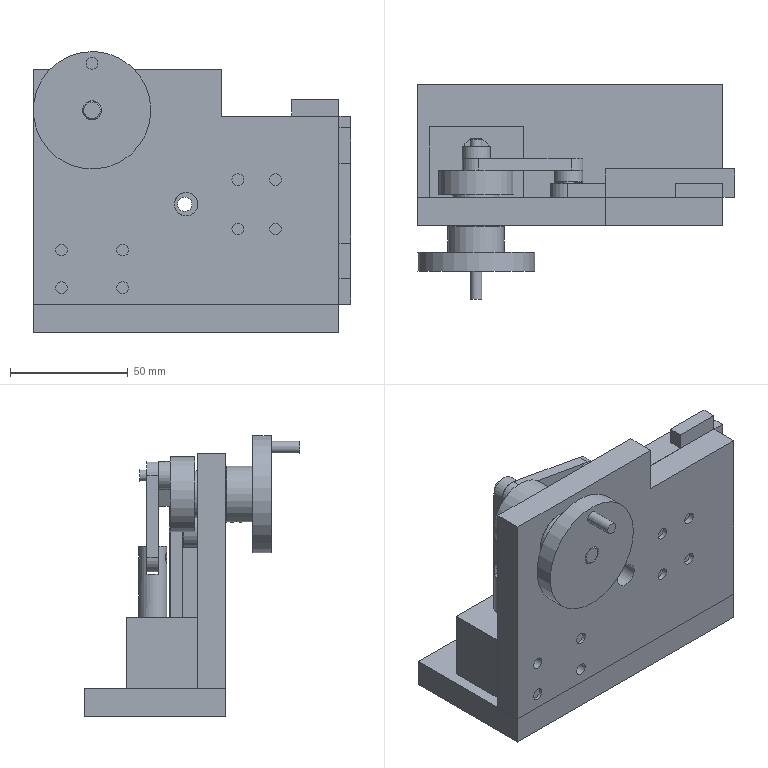Assembly | NX | mm | 27 component files | 27 solids | 262 faces | box 135 x 91.5 x 119.5 mm | volume 362094 mm3 | plane 174 | cylinder 82 | cone 6 | commonest cylinder face diameters 5 x36 12 x9 5.5 x8 10 x7 5.1 x6 8.28 x4 8 x2 6.1 x2
Bill of materials:
unnamed part 1 | 1 |  | Rectangular plate-like block with a stepped profile: raised rails/tabs and rectangular notches along its edges, a rectangular recess on one side, and four round holes in a 2x2 pattern on one region of the face.
unnamed part 2 | 1 |  | Thin flat plate of uniform thickness. One long edge is straight and the opposite edge has two V-shaped notches, giving it a sawtooth-like outline.
unnamed part 3 | 6 |  | Plain solid cylinder (round rod segment) with flat ends.
unnamed part 4 | 2 |  | Stepped cylindrical pin: a short, larger-diameter cylindrical head joined coaxially to a longer, smaller-diameter cylindrical shaft, with a flat shoulder between them.
unnamed part 5 | 1 |  | Rectangular block with one larger round hole through one face and four smaller round holes in a rectangular pattern on an adjacent face.
unnamed part 6 | 1 |  | Flanged disc: a large thin circular flange with a smaller coaxial cylindrical boss on one side. It has a central round through hole and one smaller round hole offset near the edge of the flange.
unnamed part 7 | 2 |  | Flat bar of uniform thickness with one semicircular rounded end containing a round through hole. The opposite end is pointed (chevron-shaped).
unnamed part 8 | 3 |  | Plain solid cylinder with flat ends, relatively short and wide compared with unnamed part 3.
unnamed part 9 | 1 |  | Cylinder with a conical pointed top and a rectangular slot cut into the bottom edge on one side.
unnamed part 10 | 1 |  | Flat plate of uniform thickness with a stepped outline: a rectangular portion is cut away at one corner. It has two larger round holes and two groups of four smaller round holes, each group arranged in a square or rectangular pattern.
unnamed part 11 | 1 |  | Cylindrical pin with a fork-like slotted end: a straight slot across one end forms two prongs, and a round cross hole passes through the prongs perpendicular to the slot. The slotted end region appears to have a slightly reduced outer diameter.
unnamed part 12 | 1 |  | Rectangular flat plate of uniform thickness with one larger round hole near one end and two smaller round holes spaced along one long edge.
unnamed part 13 | 1 |  | Long, narrow flat bar with one fully rounded end and one square end. It has a round hole near the rounded end, an elongated slot below that, a second round hole further down, and an open-ended slot cut into the square end, which leaves two prongs.
unnamed part 14 | 1 |  | Round, turned-style stepped part. It has a large disc-shaped head, a thin raised ring (boss) on one face of the head, a medium-diameter shank, and a smaller pin with a chamfered end. A small through-hole sits off-centre in the head.
unnamed part 15 | 1 |  | Flat link plate with fully rounded ends (stadium/obround outline) and one round through-hole near each end. The hole at one end looks larger than the hole at the other.
unnamed part 16 | 2 |  | Headed cylindrical pin: a long plain round shaft with a short cylindrical head of larger diameter at one end. Both ends appear flat.
unnamed part 17 | 1 |  | Flat link plate with fully rounded ends (obround outline) and two equal-sized round through-holes, one centred in each rounded end.
Mates:
1. touch align | groove_guide_block 1 face | vertical_plate 1 face
2. touch align | groove_guide_block 1 edge | vertical_plate 1 edge
3. concentric | groove_guide_block 1 edge | vertical_plate 1 edge
4. fix | vertical_plate 1 component
5. concentric | short_link 1 edge | slide_rod 1 edge
6. fix | round_guide_block 1 component
7. parallel | long_link 1 face | bi_link 1 face
8. concentric | long_link 1 edge | bi_link 1 edge
9. fix | eccentric_wheel 1 component
10. concentric | long_link 1 edge | eccentric_wheel 1 edge
11. touch align | handwheel 1 face | eccentric_wheel 1 face
12. concentric | eccentric_wheel 1 edge | handwheel 1 edge
13. touch align | M5x6 1 face | eccentric_wheel 1 face
14. distance | M5x6 1 face | eccentric_wheel 1 face
15. touch align | round_guide_block 1 face | hex_screw_M5_35 1 face
16. concentric | round_guide_block 1 edge | hex_screw_M5_35 1 edge
17. touch align | hex_screw_M5_35 2 face | round_guide_block 1 face
18. concentric | round_guide_block 1 edge | hex_screw_M5_35 2 edge
19. touch align | hex_screw_M5_16 2 face | groove_guide_block 1 face
20. touch align | hex_screw_M5_16 1 face | groove_guide_block 1 face
21. concentric | hex_screw_M5_16 2 edge | groove_guide_block 1 edge
22. concentric | hex_screw_M5_16 1 edge | groove_guide_block 1 edge
23. distance | vertical_plate 1 edge | dowel_pin_5_20 4 face
24. distance | dowel_pin_5_20 5 face | vertical_plate 1 face
25. touch align | vertical_plate 1 face | dowel_pin_5_20 3 face
26. touch align | vertical_plate 1 face | dowel_pin_5_20 2 face
27. concentric | dowel_pin_5_20 3 edge | round_guide_block 1 edge
28. concentric | dowel_pin_5_20 2 edge | round_guide_block 1 edge
29. touch align | dowel_pin_5_12 3 face | slide_rod 1 face
30. distance | short_link 1 face | dowel_pin_5_12 3 face
31. fix | bi_link 1 component
32. touch align | tri_slider 2 face | groove_guide_block 1 face
33. touch align | vertical_plate 1 face | V_slider 1 face
34. touch align | V_slider 1 face | groove_guide_block 1 face
35. fix | tri_slider 1 component
36. distance | V_slider 1 face | groove_guide_block 1 face
37. concentric | dowel_pin_5_12 1 edge | tri_slider 1 edge
38. concentric | dowel_pin_5_12 2 edge | tri_slider 2 edge
39. concentric | dowel_pin_5_20 1 edge | handwheel 1 edge